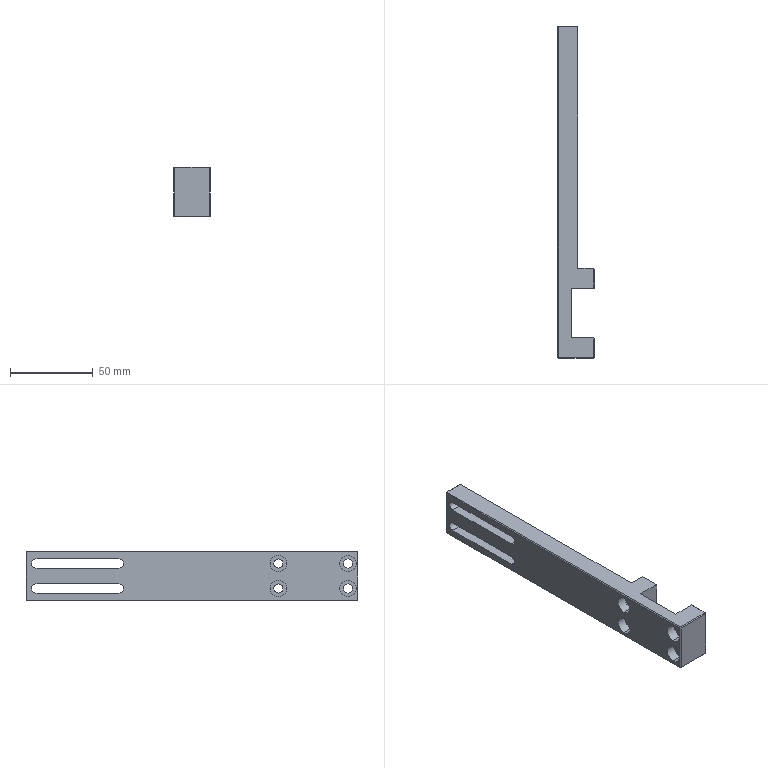Component | SolidWorks | XM-WST05-2001-1 | 1 solid | 60 faces | box 22 x 200 x 30 mm | volume 65011 mm3 | plane 40 | cylinder 20 | commonest cylinder face diameters 5.5 x12 10 x8
build123d program:
from build123d import *

# Parameters (mm, degrees)
SKETCH1_W                                            = 200
SKETCH1_H                                            = 30
BOSS_EXTRUDE1_DEPTH                                  = 22
SKETCH2_W                                            = 30
SKETCH2_H                                            = 14
CUT_EXTRUDE1_DEPTH                                   = 107.696
SKETCH3_W                                            = 146
SKETCH3_H                                            = 10
CUT_EXTRUDE2_DEPTH                                   = 107.696
CUT_EXTRUDE4_DEPTH                                   = 104.484
CHAMFER1_SIZE                                        = 0.5
HOLE_SIZE_ACCORDING_TO_HEXAGON_SOCKET_HE_D           = 5.5
HOLE_SIZE_ACCORDING_TO_HEXAGON_SOCKET_HE_CBORE_D     = 10
HOLE_SIZE_ACCORDING_TO_HEXAGON_SOCKET_HE_CBORE_DEPTH = 5.7


with BuildPart() as part:
    # Sketch1 → Boss-Extrude1 (new body)
    with BuildSketch(Plane(origin=(0, 0, 0), x_dir=(1, 0, 0), z_dir=(0, 1, 0))):
        Rectangle(SKETCH1_W, SKETCH1_H)
    extrude(amount=BOSS_EXTRUDE1_DEPTH)

    # Sketch2 → Cut-Extrude1 (cut, through all)
    with BuildSketch(Plane.XY.offset(15)):
        with Locations((73, 15)):
            Rectangle(SKETCH2_W, SKETCH2_H)
    extrude(amount=-CUT_EXTRUDE1_DEPTH, mode=Mode.SUBTRACT)

    # Sketch3 → Cut-Extrude2 (cut, through all)
    with BuildSketch(Plane.XY.offset(15)):
        with Locations((-27, 17)):
            Rectangle(SKETCH3_W, SKETCH3_H)
    extrude(amount=-CUT_EXTRUDE2_DEPTH, mode=Mode.SUBTRACT)

    # Sketch5 → Cut-Extrude4 (cut, through all)
    with BuildSketch(Plane.XZ):
        with BuildLine():
            Line((-94, 10.25), (-44, 10.25))
            ThreePointArc((-44, 10.25), (-41.25, 7.5), (-44, 4.75))
            Line((-44, 4.75), (-94, 4.75))
            ThreePointArc((-94, 4.75), (-96.75, 7.5), (-94, 10.25))
        make_face()
        with BuildLine():
            Line((-94, -10.25), (-44, -10.25))
            ThreePointArc((-44, -10.25), (-41.25, -7.5), (-44, -4.75))
            Line((-44, -4.75), (-94, -4.75))
            ThreePointArc((-94, -4.75), (-96.75, -7.5), (-94, -10.25))
        make_face()
    extrude(amount=-CUT_EXTRUDE4_DEPTH, mode=Mode.SUBTRACT)

    # Chamfer1
    chamfer1_edges = [part.edges().sort_by_distance(p)[0] for p in [
        (100, 22, 0),
        (94, 22, -15),
        (94, 22, 15),
        (52, 22, -15),
        (-100, 6, -15),
        (52, 22, 15),
        (-100, 6, 15),
        (46, 22, 0),
        (0, 0, -15),
        (100, 0, 0),
        (0, 0, 15),
        (-100, 0, 0),
        (100, 11, -15),
        (100, 11, 15),
    ]]
    chamfer(chamfer1_edges, length=CHAMFER1_SIZE)

    # Hole Size according to Hexagon Socket He (through all)
    with Locations(Plane(origin=(0, 0, 0), x_dir=(-1, 0, 0), z_dir=(0, -1, 0))):
        with Locations((-94, 7.5), (-52, 7.5), (-52, -7.5), (-94, -7.5)):
            CounterBoreHole(HOLE_SIZE_ACCORDING_TO_HEXAGON_SOCKET_HE_D / 2, HOLE_SIZE_ACCORDING_TO_HEXAGON_SOCKET_HE_CBORE_D / 2, HOLE_SIZE_ACCORDING_TO_HEXAGON_SOCKET_HE_CBORE_DEPTH)


solid = part.part

# Placed as in the assembly
solid = solid.moved(Location((-177.071, 121.669, 455.899), (0, 0, -90)))